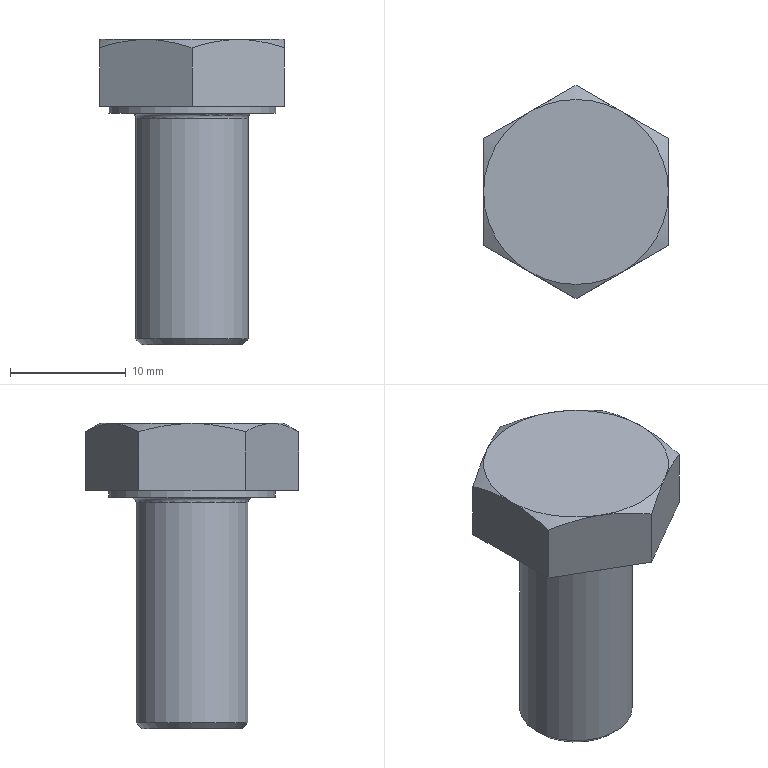Component | NX | GB-T5782-2000_M10X20 | 1 solid | 20 faces | volume 2865 mm3 | plane 10 | cone 7 | cylinder 2 | torus 1 | commonest cylinder face diameters 14.47 x1 9.732 x1